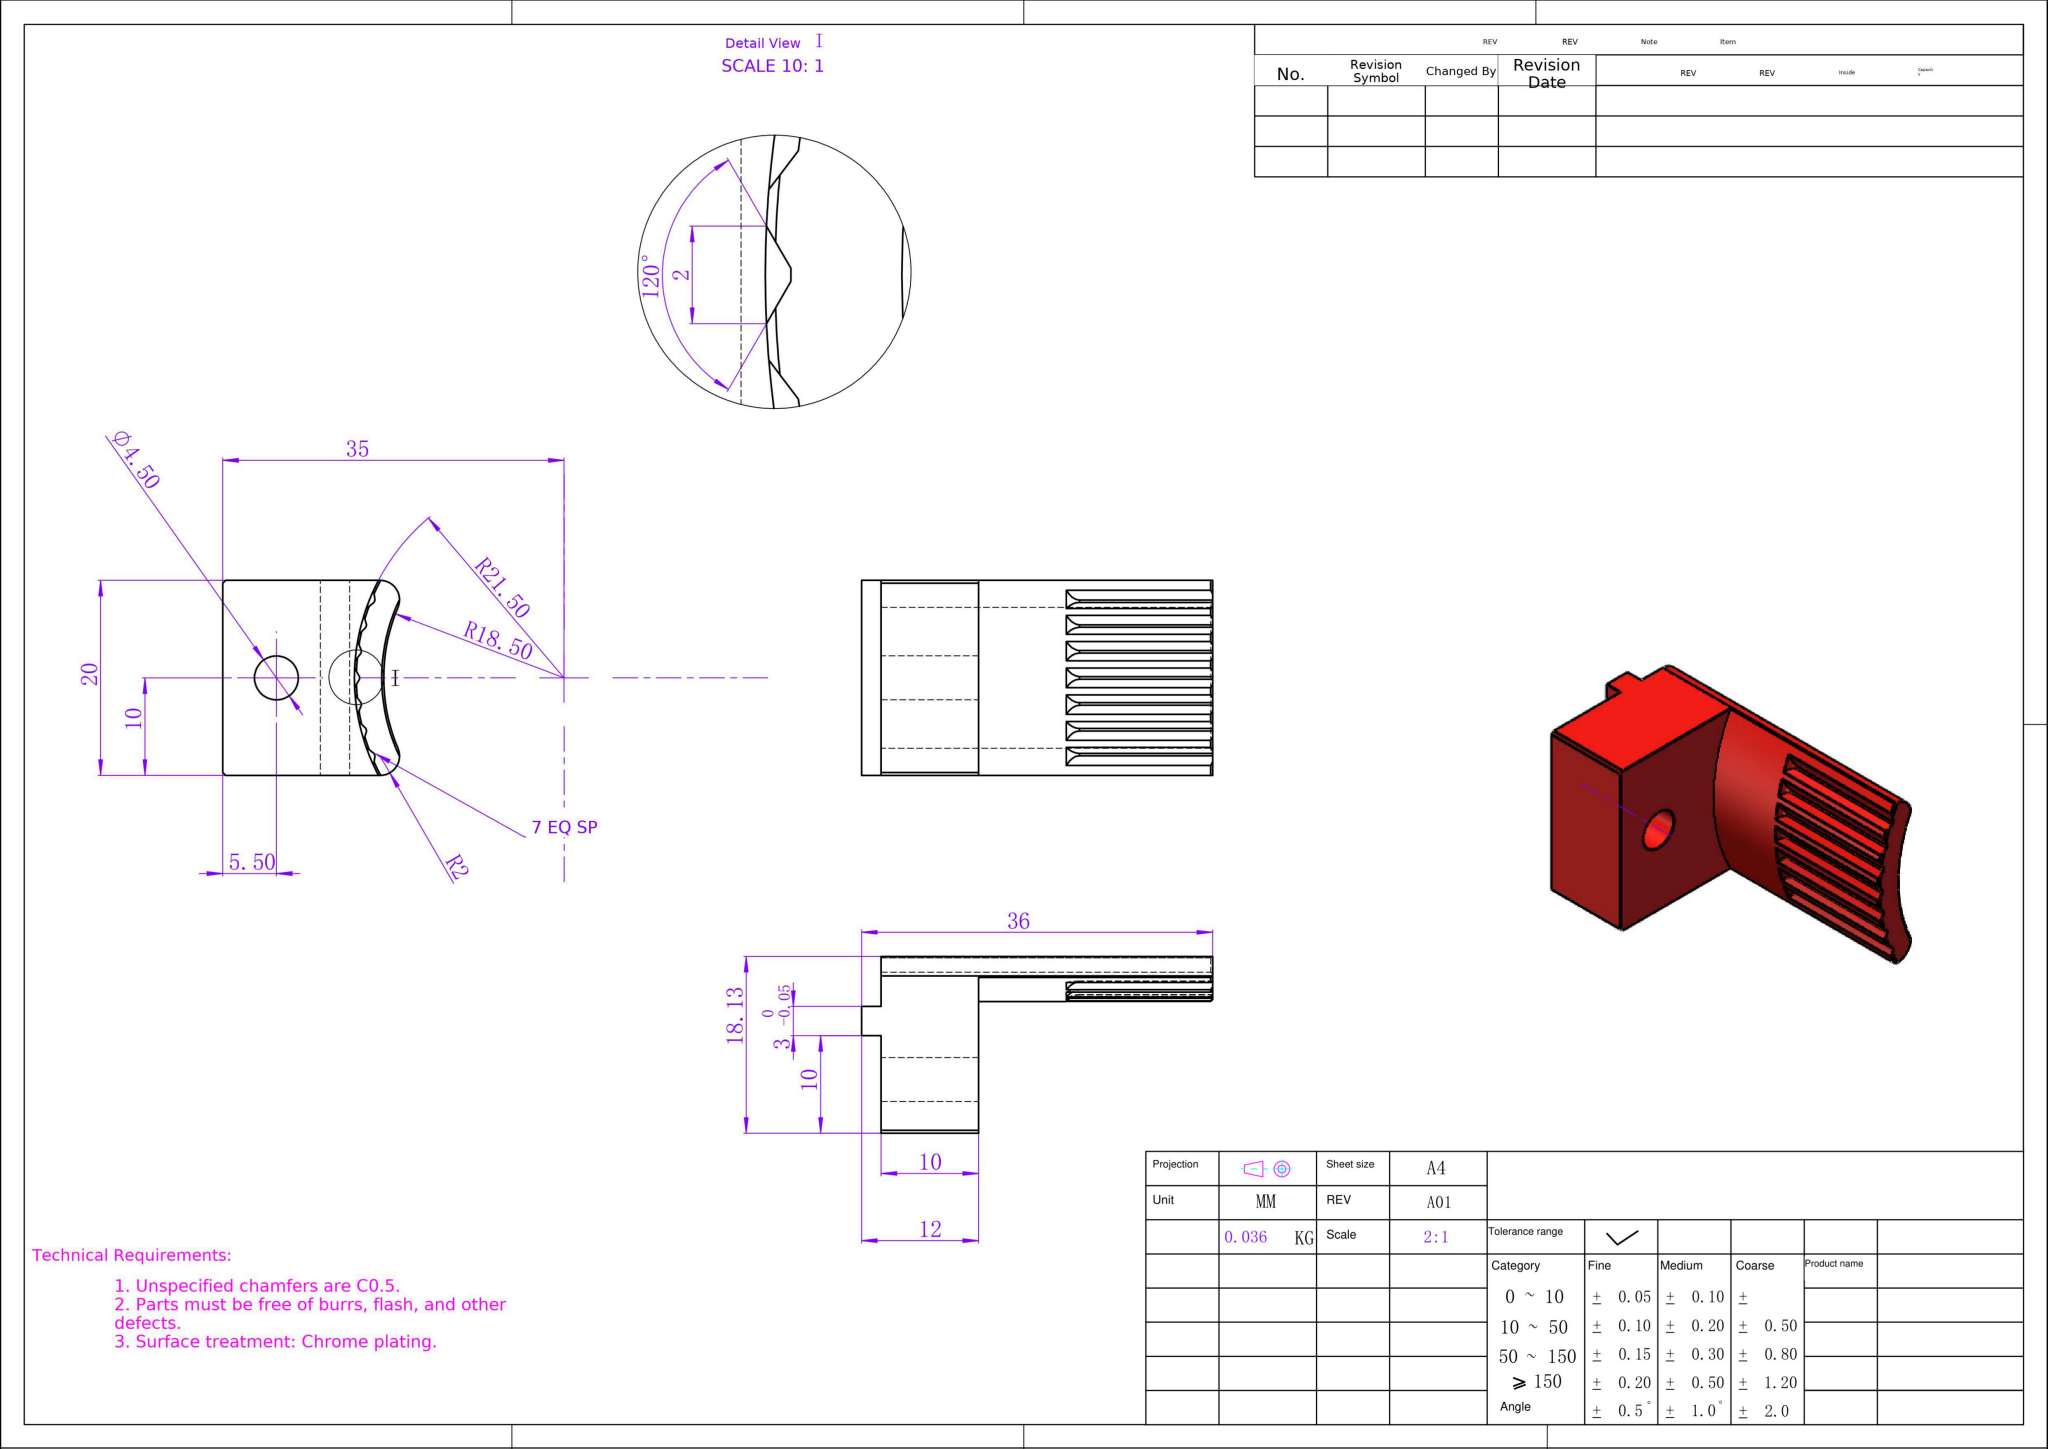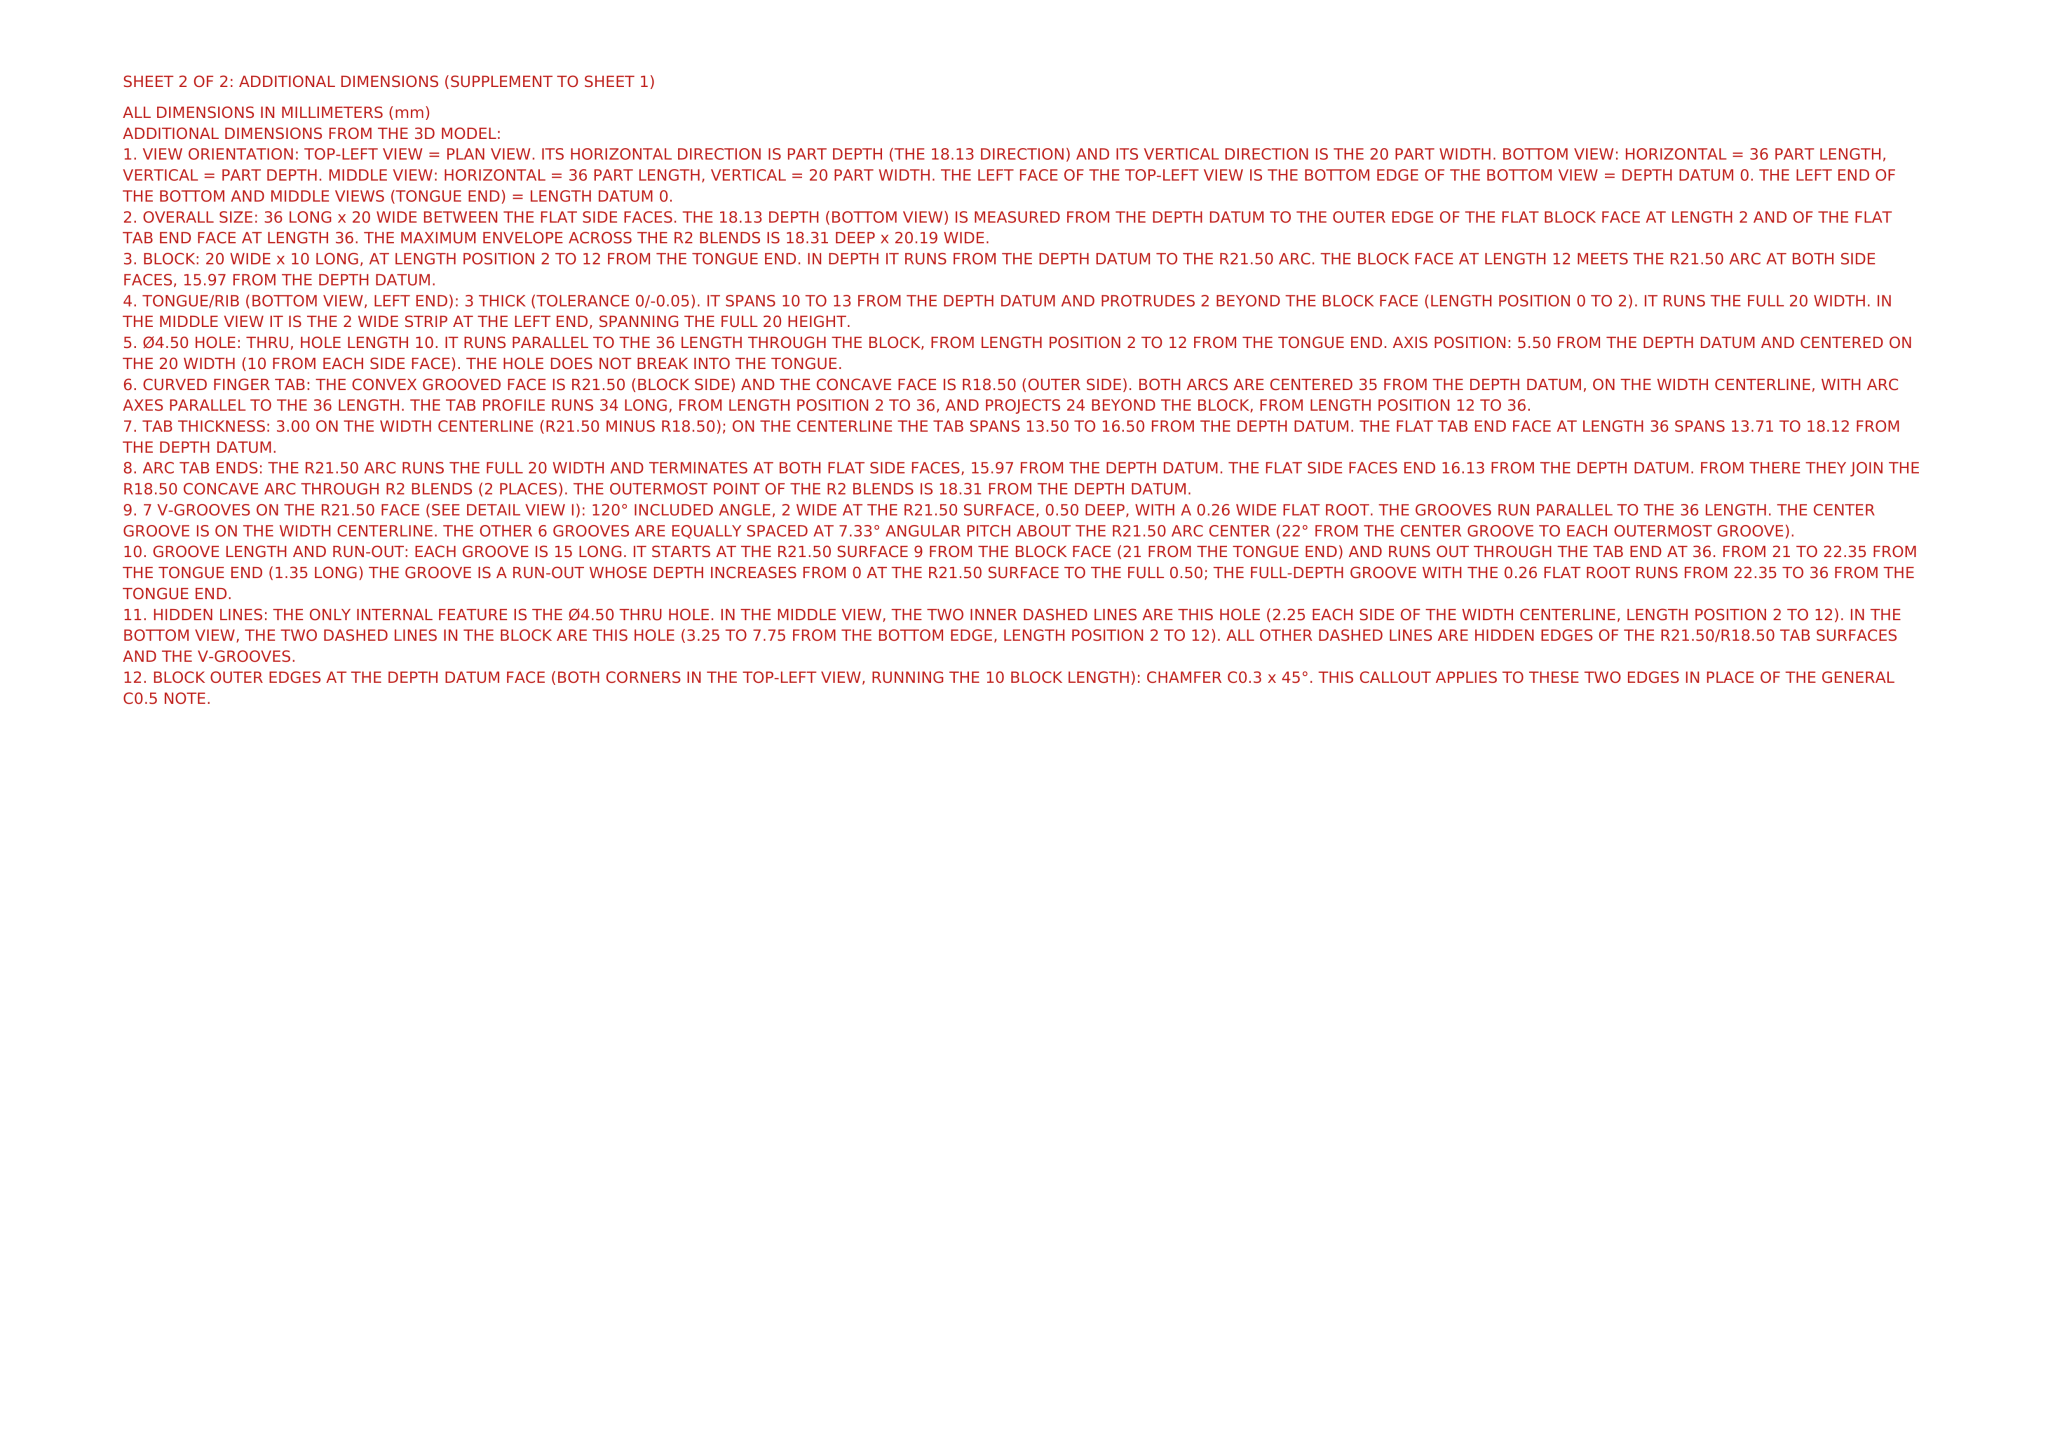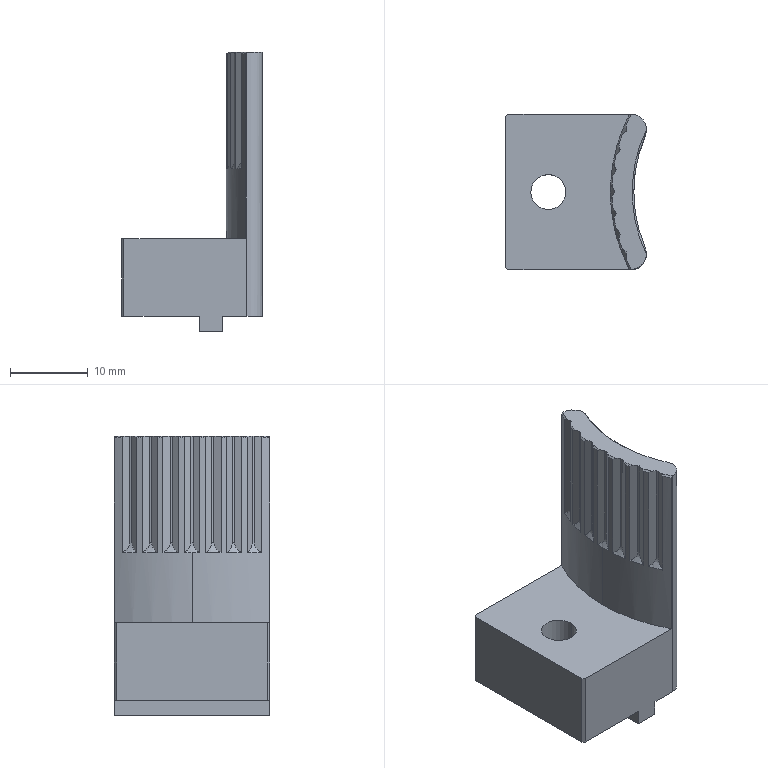Part | NX | mm | 1 solid | 57 faces | box 18.13 x 20 x 36 mm | volume 4735 mm3 | plane 33 | cone 9 | cylinder 8 | spline 7 | commonest cylinder face diameters 4.5 x2 43 x2 37 x2 4 x2